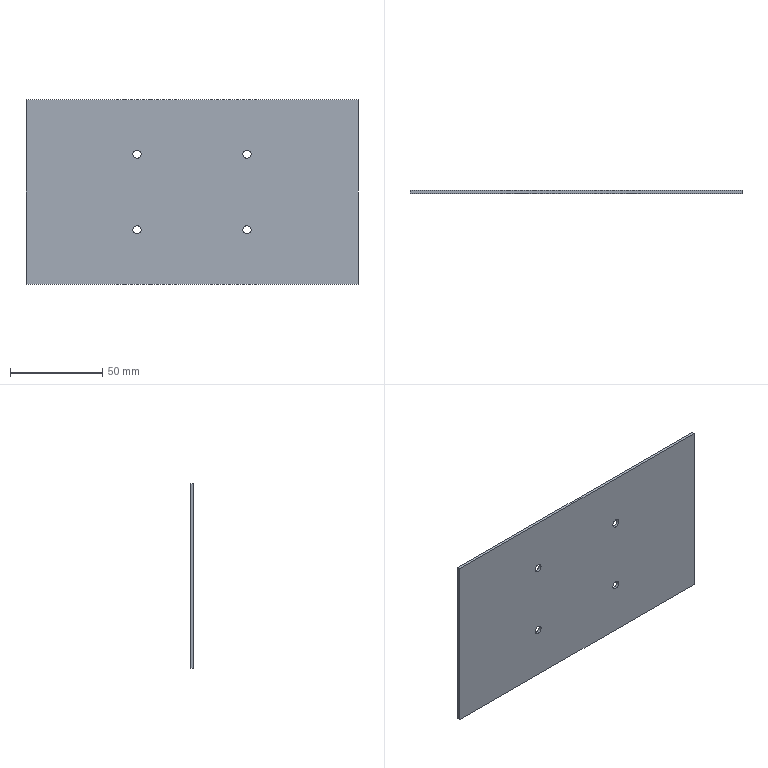Component | SolidWorks | CopperGasket-1 | 1 solid | 14 faces | box 180 x 1.5 x 100.27 mm | volume 26975 mm3 | cylinder 8 | plane 6 | commonest cylinder face diameters 4.542 x8
build123d program:
from build123d import *

# Parameters (mm, degrees)
SKETCH1_W               = 100.269
SKETCH1_H               = 180
BOSS_EXTRUDE1_DEPTH     = 1.5
SKETCH3_W               = 55.775
SKETCH3_H               = 106
BOSS_EXTRUDE2_DEPTH     = 1.5
CUT_EXTRUDE1_DEPTH      = 158.947
CUT_EXTRUDE1_DEPTH_BACK = 158.947
SKETCH2_R               = 2.271


with BuildPart() as part:
    # Sketch1 → Boss-Extrude1 (new body)
    with BuildSketch(Plane.XY):
        with Locations((0, -59.772)):
            Rectangle(SKETCH1_W, SKETCH1_H)
    extrude(amount=BOSS_EXTRUDE1_DEPTH)


with BuildPart() as body_2:
    # Sketch3 → Boss-Extrude2 (new body)
    with BuildSketch(Plane.XY.offset(1.5)):
        with Locations((0, -53)):
            Rectangle(SKETCH3_W, SKETCH3_H)
    extrude(amount=-BOSS_EXTRUDE2_DEPTH)


with BuildPart() as cut_extrude1_tool:
    # Sketch2 → Cut-Extrude1 (new, two sides: drawn at the far end of the back side and taken through both)
    with BuildSketch(Plane.XY.offset(1.5).offset(-CUT_EXTRUDE1_DEPTH_BACK)):
        with Locations((20.473, -29.973)):
            Circle(SKETCH2_R)
        with Locations((20.473, -89.571)):
            Circle(SKETCH2_R)
        with Locations((-20.473, -29.973)):
            Circle(SKETCH2_R)
        with Locations((-20.473, -89.571)):
            Circle(SKETCH2_R)
    extrude(amount=CUT_EXTRUDE1_DEPTH + CUT_EXTRUDE1_DEPTH_BACK)


with BuildPart() as part_1:
    add(part.part)

    # Cut-Extrude1: cut by cut_extrude1_tool
    add(cut_extrude1_tool.part, mode=Mode.SUBTRACT)


with BuildPart() as body_2_1:
    add(body_2.part)

    # Cut-Extrude1: cut by cut_extrude1_tool
    add(cut_extrude1_tool.part, mode=Mode.SUBTRACT)


with BuildPart() as part_2:
    add(part_1.part)

    # Combine2: union body 2
    add(body_2_1.part)


solid = part_2.part

# Placed as in the assembly
solid = solid.moved(Location((-3, 96.74, 0), (90, 0, 90)))
STEP:
#1=CARTESIAN_POINT('',(1.062,3.75,-0.7166));
#2=VERTEX_POINT('',#1);
#3=CARTESIAN_POINT('',(1.062,3.75,-0.8954));
#4=VERTEX_POINT('',#3);
#5=CARTESIAN_POINT('',(1.062,3.75,-0.806));
#6=DIRECTION('',(0.,1.,0.));
#7=DIRECTION('',(0.,0.,-1.));
#8=AXIS2_PLACEMENT_3D('',#5,#6,#7);
#9=CIRCLE('',#8,0.08941);
#10=EDGE_CURVE('',#2,#4,#9,.T.);
#11=ORIENTED_EDGE('',*,*,#10,.F.);
#12=CARTESIAN_POINT('',(1.062,3.809,-0.7166));
#13=VERTEX_POINT('',#12);
#14=CARTESIAN_POINT('',(1.062,3.75,-0.7166));
#15=DIRECTION('',(0.,1.,0.));
#16=VECTOR('',#15,39.37);
#17=LINE('',#14,#16);
#18=EDGE_CURVE('',#2,#13,#17,.T.);
#19=ORIENTED_EDGE('',*,*,#18,.T.);
#20=CARTESIAN_POINT('',(1.062,3.809,-0.8954));
#21=VERTEX_POINT('',#20);
#22=CARTESIAN_POINT('',(1.062,3.809,-0.7166));
#23=CARTESIAN_POINT('',(1.074,3.809,-0.7166));
#24=CARTESIAN_POINT('',(1.085,3.809,-0.7189));
#25=CARTESIAN_POINT('',(1.107,3.809,-0.7279));
#26=CARTESIAN_POINT('',(1.117,3.809,-0.7345));
#27=CARTESIAN_POINT('',(1.133,3.809,-0.7511));
#28=CARTESIAN_POINT('',(1.14,3.809,-0.761));
#29=CARTESIAN_POINT('',(1.149,3.809,-0.7826));
#30=CARTESIAN_POINT('',(1.151,3.809,-0.7943));
#31=CARTESIAN_POINT('',(1.151,3.809,-0.8177));
#32=CARTESIAN_POINT('',(1.149,3.809,-0.8294));
#33=CARTESIAN_POINT('',(1.14,3.809,-0.8511));
#34=CARTESIAN_POINT('',(1.133,3.809,-0.861));
#35=CARTESIAN_POINT('',(1.117,3.809,-0.8775));
#36=CARTESIAN_POINT('',(1.107,3.809,-0.8842));
#37=CARTESIAN_POINT('',(1.085,3.809,-0.8931));
#38=CARTESIAN_POINT('',(1.074,3.809,-0.8954));
#39=CARTESIAN_POINT('',(1.062,3.809,-0.8954));
#40=B_SPLINE_CURVE_WITH_KNOTS('',3,(#22,#23,#24,#25,#26,#27,#28,#29,#30,#31,#32,#33,#34,#35,#36,#37,#38,#39),.UNSPECIFIED.,.F.,.F.,(4,2,2,2,2,2,2,2,4),(0.5,0.5625,0.625,0.6875,0.75,0.8125,0.875,0.9375,1.),.UNSPECIFIED.);
#41=EDGE_CURVE('',#13,#21,#40,.T.);
#42=ORIENTED_EDGE('',*,*,#41,.T.);
#43=CARTESIAN_POINT('',(1.062,3.75,-0.8954));
#44=DIRECTION('',(0.,1.,0.));
#45=VECTOR('',#44,39.37);
#46=LINE('',#43,#45);
#47=EDGE_CURVE('',#4,#21,#46,.T.);
#48=ORIENTED_EDGE('',*,*,#47,.F.);
#49=EDGE_LOOP('',(#11,#19,#42,#48));
#50=FACE_OUTER_BOUND('',#49,.T.);
#51=CARTESIAN_POINT('',(1.062,3.75,-0.806));
#52=DIRECTION('',(0.,1.,0.));
#53=DIRECTION('',(0.,0.,-1.));
#54=AXIS2_PLACEMENT_3D('',#51,#52,#53);
#55=CYLINDRICAL_SURFACE('',#54,0.08941);
#56=ADVANCED_FACE('',(#50),#55,.F.);
#57=CARTESIAN_POINT('',(3.408,3.75,-0.7166));
#58=VERTEX_POINT('',#57);
#59=CARTESIAN_POINT('',(3.408,3.75,-0.8954));
#60=VERTEX_POINT('',#59);
#61=CARTESIAN_POINT('',(3.408,3.75,-0.806));
#62=DIRECTION('',(0.,1.,0.));
#63=DIRECTION('',(0.,0.,-1.));
#64=AXIS2_PLACEMENT_3D('',#61,#62,#63);
#65=CIRCLE('',#64,0.08941);
#66=EDGE_CURVE('',#58,#60,#65,.T.);
#67=ORIENTED_EDGE('',*,*,#66,.F.);
#68=CARTESIAN_POINT('',(3.408,3.809,-0.7166));
#69=VERTEX_POINT('',#68);
#70=CARTESIAN_POINT('',(3.408,3.75,-0.7166));
#71=DIRECTION('',(0.,1.,0.));
#72=VECTOR('',#71,39.37);
#73=LINE('',#70,#72);
#74=EDGE_CURVE('',#58,#69,#73,.T.);
#75=ORIENTED_EDGE('',*,*,#74,.T.);
#76=CARTESIAN_POINT('',(3.408,3.809,-0.8954));
#77=VERTEX_POINT('',#76);
#78=CARTESIAN_POINT('',(3.408,3.809,-0.7166));
#79=CARTESIAN_POINT('',(3.42,3.809,-0.7166));
#80=CARTESIAN_POINT('',(3.432,3.809,-0.7189));
#81=CARTESIAN_POINT('',(3.453,3.809,-0.7279));
#82=CARTESIAN_POINT('',(3.463,3.809,-0.7345));
#83=CARTESIAN_POINT('',(3.48,3.809,-0.7511));
#84=CARTESIAN_POINT('',(3.486,3.809,-0.761));
#85=CARTESIAN_POINT('',(3.495,3.809,-0.7826));
#86=CARTESIAN_POINT('',(3.498,3.809,-0.7943));
#87=CARTESIAN_POINT('',(3.498,3.809,-0.8177));
#88=CARTESIAN_POINT('',(3.495,3.809,-0.8294));
#89=CARTESIAN_POINT('',(3.486,3.809,-0.8511));
#90=CARTESIAN_POINT('',(3.48,3.809,-0.861));
#91=CARTESIAN_POINT('',(3.463,3.809,-0.8775));
#92=CARTESIAN_POINT('',(3.453,3.809,-0.8842));
#93=CARTESIAN_POINT('',(3.432,3.809,-0.8931));
#94=CARTESIAN_POINT('',(3.42,3.809,-0.8954));
#95=CARTESIAN_POINT('',(3.408,3.809,-0.8954));
#96=B_SPLINE_CURVE_WITH_KNOTS('',3,(#78,#79,#80,#81,#82,#83,#84,#85,#86,#87,#88,#89,#90,#91,#92,#93,#94,#95),.UNSPECIFIED.,.F.,.F.,(4,2,2,2,2,2,2,2,4),(0.5,0.5625,0.625,0.6875,0.75,0.8125,0.875,0.9375,1.),.UNSPECIFIED.);
#97=EDGE_CURVE('',#69,#77,#96,.T.);
#98=ORIENTED_EDGE('',*,*,#97,.T.);
#99=CARTESIAN_POINT('',(3.408,3.75,-0.8954));
#100=DIRECTION('',(0.,1.,0.));
#101=VECTOR('',#100,39.37);
#102=LINE('',#99,#101);
#103=EDGE_CURVE('',#60,#77,#102,.T.);
#104=ORIENTED_EDGE('',*,*,#103,.F.);
#105=EDGE_LOOP('',(#67,#75,#98,#104));
#106=FACE_OUTER_BOUND('',#105,.T.);
#107=CARTESIAN_POINT('',(3.408,3.75,-0.806));
#108=DIRECTION('',(0.,1.,0.));
#109=DIRECTION('',(0.,0.,-1.));
#110=AXIS2_PLACEMENT_3D('',#107,#108,#109);
#111=CYLINDRICAL_SURFACE('',#110,0.08941);
#112=ADVANCED_FACE('',(#106),#111,.F.);
#113=CARTESIAN_POINT('',(1.062,3.75,0.8954));
#114=VERTEX_POINT('',#113);
#115=CARTESIAN_POINT('',(1.062,3.75,0.7166));
#116=VERTEX_POINT('',#115);
#117=CARTESIAN_POINT('',(1.062,3.75,0.806));
#118=DIRECTION('',(0.,1.,0.));
#119=DIRECTION('',(0.,0.,-1.));
#120=AXIS2_PLACEMENT_3D('',#117,#118,#119);
#121=CIRCLE('',#120,0.08941);
#122=EDGE_CURVE('',#114,#116,#121,.T.);
#123=ORIENTED_EDGE('',*,*,#122,.F.);
#124=CARTESIAN_POINT('',(1.062,3.809,0.8954));
#125=VERTEX_POINT('',#124);
#126=CARTESIAN_POINT('',(1.062,3.75,0.8954));
#127=DIRECTION('',(0.,1.,0.));
#128=VECTOR('',#127,39.37);
#129=LINE('',#126,#128);
#130=EDGE_CURVE('',#114,#125,#129,.T.);
#131=ORIENTED_EDGE('',*,*,#130,.T.);
#132=CARTESIAN_POINT('',(1.062,3.809,0.7166));
#133=VERTEX_POINT('',#132);
#134=CARTESIAN_POINT('',(1.062,3.809,0.8954));
#135=CARTESIAN_POINT('',(1.074,3.809,0.8954));
#136=CARTESIAN_POINT('',(1.085,3.809,0.8931));
#137=CARTESIAN_POINT('',(1.107,3.809,0.8842));
#138=CARTESIAN_POINT('',(1.117,3.809,0.8775));
#139=CARTESIAN_POINT('',(1.133,3.809,0.861));
#140=CARTESIAN_POINT('',(1.14,3.809,0.8511));
#141=CARTESIAN_POINT('',(1.149,3.809,0.8294));
#142=CARTESIAN_POINT('',(1.151,3.809,0.8177));
#143=CARTESIAN_POINT('',(1.151,3.809,0.7943));
#144=CARTESIAN_POINT('',(1.149,3.809,0.7826));
#145=CARTESIAN_POINT('',(1.14,3.809,0.761));
#146=CARTESIAN_POINT('',(1.133,3.809,0.7511));
#147=CARTESIAN_POINT('',(1.117,3.809,0.7345));
#148=CARTESIAN_POINT('',(1.107,3.809,0.7279));
#149=CARTESIAN_POINT('',(1.085,3.809,0.7189));
#150=CARTESIAN_POINT('',(1.074,3.809,0.7166));
#151=CARTESIAN_POINT('',(1.062,3.809,0.7166));
#152=B_SPLINE_CURVE_WITH_KNOTS('',3,(#134,#135,#136,#137,#138,#139,#140,#141,#142,#143,#144,#145,#146,#147,#148,#149,#150,#151),.UNSPECIFIED.,.F.,.F.,(4,2,2,2,2,2,2,2,4),(0.5,0.5625,0.625,0.6875,0.75,0.8125,0.875,0.9375,1.),.UNSPECIFIED.);
#153=EDGE_CURVE('',#125,#133,#152,.T.);
#154=ORIENTED_EDGE('',*,*,#153,.T.);
#155=CARTESIAN_POINT('',(1.062,3.75,0.7166));
#156=DIRECTION('',(0.,1.,0.));
#157=VECTOR('',#156,39.37);
#158=LINE('',#155,#157);
#159=EDGE_CURVE('',#116,#133,#158,.T.);
#160=ORIENTED_EDGE('',*,*,#159,.F.);
#161=EDGE_LOOP('',(#123,#131,#154,#160));
#162=FACE_OUTER_BOUND('',#161,.T.);
#163=CARTESIAN_POINT('',(1.062,3.75,0.806));
#164=DIRECTION('',(0.,1.,0.));
#165=DIRECTION('',(0.,0.,-1.));
#166=AXIS2_PLACEMENT_3D('',#163,#164,#165);
#167=CYLINDRICAL_SURFACE('',#166,0.08941);
#168=ADVANCED_FACE('',(#162),#167,.F.);
#169=CARTESIAN_POINT('',(3.408,3.75,0.8954));
#170=VERTEX_POINT('',#169);
#171=CARTESIAN_POINT('',(3.408,3.75,0.7166));
#172=VERTEX_POINT('',#171);
#173=CARTESIAN_POINT('',(3.408,3.75,0.806));
#174=DIRECTION('',(0.,1.,0.));
#175=DIRECTION('',(0.,0.,-1.));
#176=AXIS2_PLACEMENT_3D('',#173,#174,#175);
#177=CIRCLE('',#176,0.08941);
#178=EDGE_CURVE('',#170,#172,#177,.T.);
#179=ORIENTED_EDGE('',*,*,#178,.F.);
#180=CARTESIAN_POINT('',(3.408,3.809,0.8954));
#181=VERTEX_POINT('',#180);
#182=CARTESIAN_POINT('',(3.408,3.75,0.8954));
#183=DIRECTION('',(0.,1.,0.));
#184=VECTOR('',#183,39.37);
#185=LINE('',#182,#184);
#186=EDGE_CURVE('',#170,#181,#185,.T.);
#187=ORIENTED_EDGE('',*,*,#186,.T.);
#188=CARTESIAN_POINT('',(3.408,3.809,0.7166));
#189=VERTEX_POINT('',#188);
#190=CARTESIAN_POINT('',(3.408,3.809,0.8954));
#191=CARTESIAN_POINT('',(3.42,3.809,0.8954));
#192=CARTESIAN_POINT('',(3.432,3.809,0.8931));
#193=CARTESIAN_POINT('',(3.453,3.809,0.8842));
#194=CARTESIAN_POINT('',(3.463,3.809,0.8775));
#195=CARTESIAN_POINT('',(3.48,3.809,0.861));
#196=CARTESIAN_POINT('',(3.486,3.809,0.8511));
#197=CARTESIAN_POINT('',(3.495,3.809,0.8294));
#198=CARTESIAN_POINT('',(3.498,3.809,0.8177));
#199=CARTESIAN_POINT('',(3.498,3.809,0.7943));
#200=CARTESIAN_POINT('',(3.495,3.809,0.7826));
#201=CARTESIAN_POINT('',(3.486,3.809,0.761));
#202=CARTESIAN_POINT('',(3.48,3.809,0.7511));
#203=CARTESIAN_POINT('',(3.463,3.809,0.7345));
#204=CARTESIAN_POINT('',(3.453,3.809,0.7279));
#205=CARTESIAN_POINT('',(3.432,3.809,0.7189));
#206=CARTESIAN_POINT('',(3.42,3.809,0.7166));
#207=CARTESIAN_POINT('',(3.408,3.809,0.7166));
#208=B_SPLINE_CURVE_WITH_KNOTS('',3,(#190,#191,#192,#193,#194,#195,#196,#197,#198,#199,#200,#201,#202,#203,#204,#205,#206,#207),.UNSPECIFIED.,.F.,.F.,(4,2,2,2,2,2,2,2,4),(0.5,0.5625,0.625,0.6875,0.75,0.8125,0.875,0.9375,1.),.UNSPECIFIED.);
#209=EDGE_CURVE('',#181,#189,#208,.T.);
#210=ORIENTED_EDGE('',*,*,#209,.T.);
#211=CARTESIAN_POINT('',(3.408,3.75,0.7166));
#212=DIRECTION('',(0.,1.,0.));
#213=VECTOR('',#212,39.37);
#214=LINE('',#211,#213);
#215=EDGE_CURVE('',#172,#189,#214,.T.);
#216=ORIENTED_EDGE('',*,*,#215,.F.);
#217=EDGE_LOOP('',(#179,#187,#210,#216));
#218=FACE_OUTER_BOUND('',#217,.T.);
#219=CARTESIAN_POINT('',(3.408,3.75,0.806));
#220=DIRECTION('',(0.,1.,0.));
#221=DIRECTION('',(0.,0.,-1.));
#222=AXIS2_PLACEMENT_3D('',#219,#220,#221);
#223=CYLINDRICAL_SURFACE('',#222,0.08941);
#224=ADVANCED_FACE('',(#218),#223,.F.);
#225=CARTESIAN_POINT('',(5.778,3.75,-1.974));
#226=VERTEX_POINT('',#225);
#227=CARTESIAN_POINT('',(-1.308,3.75,-1.974));
#228=VERTEX_POINT('',#227);
#229=CARTESIAN_POINT('',(5.778,3.75,-1.974));
#230=DIRECTION('',(-1.,-0.,0.));
#231=VECTOR('',#230,39.37);
#232=LINE('',#229,#231);
#233=EDGE_CURVE('',#226,#228,#232,.T.);
#234=ORIENTED_EDGE('',*,*,#233,.T.);
#235=CARTESIAN_POINT('',(-1.308,3.809,-1.974));
#236=VERTEX_POINT('',#235);
#237=CARTESIAN_POINT('',(-1.308,3.809,-1.974));
#238=DIRECTION('',(0.,-1.,-0.));
#239=VECTOR('',#238,39.37);
#240=LINE('',#237,#239);
#241=EDGE_CURVE('',#236,#228,#240,.T.);
#242=ORIENTED_EDGE('',*,*,#241,.F.);
#243=CARTESIAN_POINT('',(5.778,3.809,-1.974));
#244=VERTEX_POINT('',#243);
#245=CARTESIAN_POINT('',(5.778,3.809,-1.974));
#246=DIRECTION('',(-1.,-0.,0.));
#247=VECTOR('',#246,39.37);
#248=LINE('',#245,#247);
#249=EDGE_CURVE('',#244,#236,#248,.T.);
#250=ORIENTED_EDGE('',*,*,#249,.F.);
#251=CARTESIAN_POINT('',(5.778,3.809,-1.974));
#252=DIRECTION('',(0.,-1.,-0.));
#253=VECTOR('',#252,39.37);
#254=LINE('',#251,#253);
#255=EDGE_CURVE('',#244,#226,#254,.T.);
#256=ORIENTED_EDGE('',*,*,#255,.T.);
#257=EDGE_LOOP('',(#234,#242,#250,#256));
#258=FACE_OUTER_BOUND('',#257,.T.);
#259=CARTESIAN_POINT('',(5.778,3.809,-1.974));
#260=DIRECTION('',(0.,-0.,1.));
#261=DIRECTION('',(1.,0.,-0.));
#262=AXIS2_PLACEMENT_3D('',#259,#260,#261);
#263=PLANE('',#262);
#264=ADVANCED_FACE('',(#258),#263,.F.);
#265=CARTESIAN_POINT('',(-1.308,3.75,1.974));
#266=VERTEX_POINT('',#265);
#267=CARTESIAN_POINT('',(-1.308,3.75,-1.974));
#268=DIRECTION('',(0.,-0.,1.));
#269=VECTOR('',#268,39.37);
#270=LINE('',#267,#269);
#271=EDGE_CURVE('',#228,#266,#270,.T.);
#272=ORIENTED_EDGE('',*,*,#271,.T.);
#273=CARTESIAN_POINT('',(-1.308,3.809,1.974));
#274=VERTEX_POINT('',#273);
#275=CARTESIAN_POINT('',(-1.308,3.809,1.974));
#276=DIRECTION('',(0.,-1.,-0.));
#277=VECTOR('',#276,39.37);
#278=LINE('',#275,#277);
#279=EDGE_CURVE('',#274,#266,#278,.T.);
#280=ORIENTED_EDGE('',*,*,#279,.F.);
#281=CARTESIAN_POINT('',(-1.308,3.809,-1.974));
#282=DIRECTION('',(0.,-0.,1.));
#283=VECTOR('',#282,39.37);
#284=LINE('',#281,#283);
#285=EDGE_CURVE('',#236,#274,#284,.T.);
#286=ORIENTED_EDGE('',*,*,#285,.F.);
#287=ORIENTED_EDGE('',*,*,#241,.T.);
#288=EDGE_LOOP('',(#272,#280,#286,#287));
#289=FACE_OUTER_BOUND('',#288,.T.);
#290=CARTESIAN_POINT('',(-1.308,3.809,-1.974));
#291=DIRECTION('',(1.,0.,-0.));
#292=DIRECTION('',(0.,-1.,-0.));
#293=AXIS2_PLACEMENT_3D('',#290,#291,#292);
#294=PLANE('',#293);
#295=ADVANCED_FACE('',(#289),#294,.F.);
#296=CARTESIAN_POINT('',(5.778,3.75,1.974));
#297=VERTEX_POINT('',#296);
#298=CARTESIAN_POINT('',(-1.308,3.75,1.974));
#299=DIRECTION('',(1.,0.,-0.));
#300=VECTOR('',#299,39.37);
#301=LINE('',#298,#300);
#302=EDGE_CURVE('',#266,#297,#301,.T.);
#303=ORIENTED_EDGE('',*,*,#302,.T.);
#304=CARTESIAN_POINT('',(5.778,3.809,1.974));
#305=VERTEX_POINT('',#304);
#306=CARTESIAN_POINT('',(5.778,3.809,1.974));
#307=DIRECTION('',(0.,-1.,-0.));
#308=VECTOR('',#307,39.37);
#309=LINE('',#306,#308);
#310=EDGE_CURVE('',#305,#297,#309,.T.);
#311=ORIENTED_EDGE('',*,*,#310,.F.);
#312=CARTESIAN_POINT('',(-1.308,3.809,1.974));
#313=DIRECTION('',(1.,0.,-0.));
#314=VECTOR('',#313,39.37);
#315=LINE('',#312,#314);
#316=EDGE_CURVE('',#274,#305,#315,.T.);
#317=ORIENTED_EDGE('',*,*,#316,.F.);
#318=ORIENTED_EDGE('',*,*,#279,.T.);
#319=EDGE_LOOP('',(#303,#311,#317,#318));
#320=FACE_OUTER_BOUND('',#319,.T.);
#321=CARTESIAN_POINT('',(-1.308,3.809,1.974));
#322=DIRECTION('',(-0.,0.,-1.));
#323=DIRECTION('',(-1.,-0.,0.));
#324=AXIS2_PLACEMENT_3D('',#321,#322,#323);
#325=PLANE('',#324);
#326=ADVANCED_FACE('',(#320),#325,.F.);
#327=CARTESIAN_POINT('',(5.778,3.75,1.974));
#328=DIRECTION('',(0.,0.,-1.));
#329=VECTOR('',#328,39.37);
#330=LINE('',#327,#329);
#331=EDGE_CURVE('',#297,#226,#330,.T.);
#332=ORIENTED_EDGE('',*,*,#331,.T.);
#333=ORIENTED_EDGE('',*,*,#255,.F.);
#334=CARTESIAN_POINT('',(5.778,3.809,1.974));
#335=DIRECTION('',(0.,0.,-1.));
#336=VECTOR('',#335,39.37);
#337=LINE('',#334,#336);
#338=EDGE_CURVE('',#305,#244,#337,.T.);
#339=ORIENTED_EDGE('',*,*,#338,.F.);
#340=ORIENTED_EDGE('',*,*,#310,.T.);
#341=EDGE_LOOP('',(#332,#333,#339,#340));
#342=FACE_OUTER_BOUND('',#341,.T.);
#343=CARTESIAN_POINT('',(5.778,3.809,1.974));
#344=DIRECTION('',(-1.,-0.,0.));
#345=DIRECTION('',(0.,1.,0.));
#346=AXIS2_PLACEMENT_3D('',#343,#344,#345);
#347=PLANE('',#346);
#348=ADVANCED_FACE('',(#342),#347,.F.);
#349=CARTESIAN_POINT('',(1.062,3.809,-0.8954));
#350=CARTESIAN_POINT('',(1.05,3.809,-0.8954));
#351=CARTESIAN_POINT('',(1.039,3.809,-0.8931));
#352=CARTESIAN_POINT('',(1.017,3.809,-0.8842));
#353=CARTESIAN_POINT('',(1.007,3.809,-0.8775));
#354=CARTESIAN_POINT('',(0.9904,3.809,-0.861));
#355=CARTESIAN_POINT('',(0.9838,3.809,-0.8511));
#356=CARTESIAN_POINT('',(0.9748,3.809,-0.8294));
#357=CARTESIAN_POINT('',(0.9725,3.809,-0.8177));
#358=CARTESIAN_POINT('',(0.9725,3.809,-0.7943));
#359=CARTESIAN_POINT('',(0.9748,3.809,-0.7826));
#360=CARTESIAN_POINT('',(0.9838,3.809,-0.761));
#361=CARTESIAN_POINT('',(0.9904,3.809,-0.7511));
#362=CARTESIAN_POINT('',(1.007,3.809,-0.7345));
#363=CARTESIAN_POINT('',(1.017,3.809,-0.7279));
#364=CARTESIAN_POINT('',(1.039,3.809,-0.7189));
#365=CARTESIAN_POINT('',(1.05,3.809,-0.7166));
#366=CARTESIAN_POINT('',(1.062,3.809,-0.7166));
#367=B_SPLINE_CURVE_WITH_KNOTS('',3,(#349,#350,#351,#352,#353,#354,#355,#356,#357,#358,#359,#360,#361,#362,#363,#364,#365,#366),.UNSPECIFIED.,.F.,.F.,(4,2,2,2,2,2,2,2,4),(0.,0.0625,0.125,0.1875,0.25,0.3125,0.375,0.4375,0.5),.UNSPECIFIED.);
#368=EDGE_CURVE('',#21,#13,#367,.T.);
#369=ORIENTED_EDGE('',*,*,#368,.F.);
#370=ORIENTED_EDGE('',*,*,#41,.F.);
#371=EDGE_LOOP('',(#369,#370));
#372=FACE_BOUND('',#371,.T.);
#373=CARTESIAN_POINT('',(3.408,3.809,-0.8954));
#374=CARTESIAN_POINT('',(3.397,3.809,-0.8954));
#375=CARTESIAN_POINT('',(3.385,3.809,-0.8931));
#376=CARTESIAN_POINT('',(3.363,3.809,-0.8842));
#377=CARTESIAN_POINT('',(3.353,3.809,-0.8775));
#378=CARTESIAN_POINT('',(3.337,3.809,-0.861));
#379=CARTESIAN_POINT('',(3.33,3.809,-0.8511));
#380=CARTESIAN_POINT('',(3.321,3.809,-0.8294));
#381=CARTESIAN_POINT('',(3.319,3.809,-0.8177));
#382=CARTESIAN_POINT('',(3.319,3.809,-0.7943));
#383=CARTESIAN_POINT('',(3.321,3.809,-0.7826));
#384=CARTESIAN_POINT('',(3.33,3.809,-0.761));
#385=CARTESIAN_POINT('',(3.337,3.809,-0.7511));
#386=CARTESIAN_POINT('',(3.353,3.809,-0.7345));
#387=CARTESIAN_POINT('',(3.363,3.809,-0.7279));
#388=CARTESIAN_POINT('',(3.385,3.809,-0.7189));
#389=CARTESIAN_POINT('',(3.397,3.809,-0.7166));
#390=CARTESIAN_POINT('',(3.408,3.809,-0.7166));
#391=B_SPLINE_CURVE_WITH_KNOTS('',3,(#373,#374,#375,#376,#377,#378,#379,#380,#381,#382,#383,#384,#385,#386,#387,#388,#389,#390),.UNSPECIFIED.,.F.,.F.,(4,2,2,2,2,2,2,2,4),(0.,0.0625,0.125,0.1875,0.25,0.3125,0.375,0.4375,0.5),.UNSPECIFIED.);
#392=EDGE_CURVE('',#77,#69,#391,.T.);
#393=ORIENTED_EDGE('',*,*,#392,.F.);
#394=ORIENTED_EDGE('',*,*,#97,.F.);
#395=EDGE_LOOP('',(#393,#394));
#396=FACE_BOUND('',#395,.T.);
#397=CARTESIAN_POINT('',(1.062,3.809,0.7166));
#398=CARTESIAN_POINT('',(1.05,3.809,0.7166));
#399=CARTESIAN_POINT('',(1.039,3.809,0.7189));
#400=CARTESIAN_POINT('',(1.017,3.809,0.7279));
#401=CARTESIAN_POINT('',(1.007,3.809,0.7345));
#402=CARTESIAN_POINT('',(0.9904,3.809,0.7511));
#403=CARTESIAN_POINT('',(0.9838,3.809,0.761));
#404=CARTESIAN_POINT('',(0.9748,3.809,0.7826));
#405=CARTESIAN_POINT('',(0.9725,3.809,0.7943));
#406=CARTESIAN_POINT('',(0.9725,3.809,0.8177));
#407=CARTESIAN_POINT('',(0.9748,3.809,0.8294));
#408=CARTESIAN_POINT('',(0.9838,3.809,0.8511));
#409=CARTESIAN_POINT('',(0.9904,3.809,0.861));
#410=CARTESIAN_POINT('',(1.007,3.809,0.8775));
#411=CARTESIAN_POINT('',(1.017,3.809,0.8842));
#412=CARTESIAN_POINT('',(1.039,3.809,0.8931));
#413=CARTESIAN_POINT('',(1.05,3.809,0.8954));
#414=CARTESIAN_POINT('',(1.062,3.809,0.8954));
#415=B_SPLINE_CURVE_WITH_KNOTS('',3,(#397,#398,#399,#400,#401,#402,#403,#404,#405,#406,#407,#408,#409,#410,#411,#412,#413,#414),.UNSPECIFIED.,.F.,.F.,(4,2,2,2,2,2,2,2,4),(0.,0.0625,0.125,0.1875,0.25,0.3125,0.375,0.4375,0.5),.UNSPECIFIED.);
#416=EDGE_CURVE('',#133,#125,#415,.T.);
#417=ORIENTED_EDGE('',*,*,#416,.F.);
#418=ORIENTED_EDGE('',*,*,#153,.F.);
#419=EDGE_LOOP('',(#417,#418));
#420=FACE_BOUND('',#419,.T.);
#421=CARTESIAN_POINT('',(3.408,3.809,0.7166));
#422=CARTESIAN_POINT('',(3.397,3.809,0.7166));
#423=CARTESIAN_POINT('',(3.385,3.809,0.7189));
#424=CARTESIAN_POINT('',(3.363,3.809,0.7279));
#425=CARTESIAN_POINT('',(3.353,3.809,0.7345));
#426=CARTESIAN_POINT('',(3.337,3.809,0.7511));
#427=CARTESIAN_POINT('',(3.33,3.809,0.761));
#428=CARTESIAN_POINT('',(3.321,3.809,0.7826));
#429=CARTESIAN_POINT('',(3.319,3.809,0.7943));
#430=CARTESIAN_POINT('',(3.319,3.809,0.8177));
#431=CARTESIAN_POINT('',(3.321,3.809,0.8294));
#432=CARTESIAN_POINT('',(3.33,3.809,0.8511));
#433=CARTESIAN_POINT('',(3.337,3.809,0.861));
#434=CARTESIAN_POINT('',(3.353,3.809,0.8775));
#435=CARTESIAN_POINT('',(3.363,3.809,0.8842));
#436=CARTESIAN_POINT('',(3.385,3.809,0.8931));
#437=CARTESIAN_POINT('',(3.397,3.809,0.8954));
#438=CARTESIAN_POINT('',(3.408,3.809,0.8954));
#439=B_SPLINE_CURVE_WITH_KNOTS('',3,(#421,#422,#423,#424,#425,#426,#427,#428,#429,#430,#431,#432,#433,#434,#435,#436,#437,#438),.UNSPECIFIED.,.F.,.F.,(4,2,2,2,2,2,2,2,4),(0.,0.0625,0.125,0.1875,0.25,0.3125,0.375,0.4375,0.5),.UNSPECIFIED.);
#440=EDGE_CURVE('',#189,#181,#439,.T.);
#441=ORIENTED_EDGE('',*,*,#440,.F.);
#442=ORIENTED_EDGE('',*,*,#209,.F.);
#443=EDGE_LOOP('',(#441,#442));
#444=FACE_BOUND('',#443,.T.);
#445=ORIENTED_EDGE('',*,*,#249,.T.);
#446=ORIENTED_EDGE('',*,*,#285,.T.);
#447=ORIENTED_EDGE('',*,*,#316,.T.);
#448=ORIENTED_EDGE('',*,*,#338,.T.);
#449=EDGE_LOOP('',(#445,#446,#447,#448));
#450=FACE_OUTER_BOUND('',#449,.T.);
#451=CARTESIAN_POINT('',(-0.1181,3.809,-0.));
#452=DIRECTION('',(0.,1.,0.));
#453=DIRECTION('',(0.,0.,-1.));
#454=AXIS2_PLACEMENT_3D('',#451,#452,#453);
#455=PLANE('',#454);
#456=ADVANCED_FACE('',(#372,#396,#420,#444,#450),#455,.T.);
#457=CARTESIAN_POINT('',(1.062,3.75,-0.806));
#458=DIRECTION('',(0.,1.,0.));
#459=DIRECTION('',(0.,0.,-1.));
#460=AXIS2_PLACEMENT_3D('',#457,#458,#459);
#461=CIRCLE('',#460,0.08941);
#462=EDGE_CURVE('',#4,#2,#461,.T.);
#463=ORIENTED_EDGE('',*,*,#462,.T.);
#464=ORIENTED_EDGE('',*,*,#10,.T.);
#465=EDGE_LOOP('',(#463,#464));
#466=FACE_BOUND('',#465,.T.);
#467=CARTESIAN_POINT('',(3.408,3.75,-0.806));
#468=DIRECTION('',(0.,1.,0.));
#469=DIRECTION('',(0.,0.,-1.));
#470=AXIS2_PLACEMENT_3D('',#467,#468,#469);
#471=CIRCLE('',#470,0.08941);
#472=EDGE_CURVE('',#60,#58,#471,.T.);
#473=ORIENTED_EDGE('',*,*,#472,.T.);
#474=ORIENTED_EDGE('',*,*,#66,.T.);
#475=EDGE_LOOP('',(#473,#474));
#476=FACE_BOUND('',#475,.T.);
#477=CARTESIAN_POINT('',(1.062,3.75,0.806));
#478=DIRECTION('',(0.,1.,0.));
#479=DIRECTION('',(0.,0.,-1.));
#480=AXIS2_PLACEMENT_3D('',#477,#478,#479);
#481=CIRCLE('',#480,0.08941);
#482=EDGE_CURVE('',#116,#114,#481,.T.);
#483=ORIENTED_EDGE('',*,*,#482,.T.);
#484=ORIENTED_EDGE('',*,*,#122,.T.);
#485=EDGE_LOOP('',(#483,#484));
#486=FACE_BOUND('',#485,.T.);
#487=CARTESIAN_POINT('',(3.408,3.75,0.806));
#488=DIRECTION('',(0.,1.,0.));
#489=DIRECTION('',(0.,0.,-1.));
#490=AXIS2_PLACEMENT_3D('',#487,#488,#489);
#491=CIRCLE('',#490,0.08941);
#492=EDGE_CURVE('',#172,#170,#491,.T.);
#493=ORIENTED_EDGE('',*,*,#492,.T.);
#494=ORIENTED_EDGE('',*,*,#178,.T.);
#495=EDGE_LOOP('',(#493,#494));
#496=FACE_BOUND('',#495,.T.);
#497=ORIENTED_EDGE('',*,*,#233,.F.);
#498=ORIENTED_EDGE('',*,*,#331,.F.);
#499=ORIENTED_EDGE('',*,*,#302,.F.);
#500=ORIENTED_EDGE('',*,*,#271,.F.);
#501=EDGE_LOOP('',(#497,#498,#499,#500));
#502=FACE_OUTER_BOUND('',#501,.T.);
#503=CARTESIAN_POINT('',(-0.1181,3.75,-0.));
#504=DIRECTION('',(0.,1.,0.));
#505=DIRECTION('',(0.,0.,-1.));
#506=AXIS2_PLACEMENT_3D('',#503,#504,#505);
#507=PLANE('',#506);
#508=ADVANCED_FACE('',(#466,#476,#486,#496,#502),#507,.F.);
#509=ORIENTED_EDGE('',*,*,#186,.F.);
#510=ORIENTED_EDGE('',*,*,#492,.F.);
#511=ORIENTED_EDGE('',*,*,#215,.T.);
#512=ORIENTED_EDGE('',*,*,#440,.T.);
#513=EDGE_LOOP('',(#509,#510,#511,#512));
#514=FACE_OUTER_BOUND('',#513,.T.);
#515=CARTESIAN_POINT('',(3.408,3.75,0.806));
#516=DIRECTION('',(0.,1.,0.));
#517=DIRECTION('',(0.,0.,-1.));
#518=AXIS2_PLACEMENT_3D('',#515,#516,#517);
#519=CYLINDRICAL_SURFACE('',#518,0.08941);
#520=ADVANCED_FACE('',(#514),#519,.F.);
#521=ORIENTED_EDGE('',*,*,#130,.F.);
#522=ORIENTED_EDGE('',*,*,#482,.F.);
#523=ORIENTED_EDGE('',*,*,#159,.T.);
#524=ORIENTED_EDGE('',*,*,#416,.T.);
#525=EDGE_LOOP('',(#521,#522,#523,#524));
#526=FACE_OUTER_BOUND('',#525,.T.);
#527=CARTESIAN_POINT('',(1.062,3.75,0.806));
#528=DIRECTION('',(0.,1.,0.));
#529=DIRECTION('',(0.,0.,-1.));
#530=AXIS2_PLACEMENT_3D('',#527,#528,#529);
#531=CYLINDRICAL_SURFACE('',#530,0.08941);
#532=ADVANCED_FACE('',(#526),#531,.F.);
#533=ORIENTED_EDGE('',*,*,#74,.F.);
#534=ORIENTED_EDGE('',*,*,#472,.F.);
#535=ORIENTED_EDGE('',*,*,#103,.T.);
#536=ORIENTED_EDGE('',*,*,#392,.T.);
#537=EDGE_LOOP('',(#533,#534,#535,#536));
#538=FACE_OUTER_BOUND('',#537,.T.);
#539=CARTESIAN_POINT('',(3.408,3.75,-0.806));
#540=DIRECTION('',(0.,1.,0.));
#541=DIRECTION('',(0.,0.,-1.));
#542=AXIS2_PLACEMENT_3D('',#539,#540,#541);
#543=CYLINDRICAL_SURFACE('',#542,0.08941);
#544=ADVANCED_FACE('',(#538),#543,.F.);
#545=ORIENTED_EDGE('',*,*,#18,.F.);
#546=ORIENTED_EDGE('',*,*,#462,.F.);
#547=ORIENTED_EDGE('',*,*,#47,.T.);
#548=ORIENTED_EDGE('',*,*,#368,.T.);
#549=EDGE_LOOP('',(#545,#546,#547,#548));
#550=FACE_OUTER_BOUND('',#549,.T.);
#551=CARTESIAN_POINT('',(1.062,3.75,-0.806));
#552=DIRECTION('',(0.,1.,0.));
#553=DIRECTION('',(0.,0.,-1.));
#554=AXIS2_PLACEMENT_3D('',#551,#552,#553);
#555=CYLINDRICAL_SURFACE('',#554,0.08941);
#556=ADVANCED_FACE('',(#550),#555,.F.);
#557=CLOSED_SHELL('',(#56,#112,#168,#224,#264,#295,#326,#348,#456,#508,#520,#532,#544,#556));
#558=MANIFOLD_SOLID_BREP('',#557);
#559=CARTESIAN_POINT('',(0.,0.,0.));
#560=DIRECTION('',(0.,0.,1.));
#561=DIRECTION('',(1.,0.,0.));
#562=AXIS2_PLACEMENT_3D('',#559,#560,#561);
#563=(LENGTH_UNIT()NAMED_UNIT(*)SI_UNIT($,.METRE.));
#564=LENGTH_MEASURE_WITH_UNIT(LENGTH_MEASURE(0.0254),#563);
#565=DIMENSIONAL_EXPONENTS(1.,0.,0.,0.,0.,0.,0.);
#566=(CONVERSION_BASED_UNIT('',#564)LENGTH_UNIT()NAMED_UNIT(#565));
#567=UNCERTAINTY_MEASURE_WITH_UNIT(LENGTH_MEASURE(0.00001),#566,'','');
#568=(NAMED_UNIT(*)PLANE_ANGLE_UNIT()SI_UNIT($,.RADIAN.));
#569=(NAMED_UNIT(*)SI_UNIT($,.STERADIAN.)SOLID_ANGLE_UNIT());
#570=(GEOMETRIC_REPRESENTATION_CONTEXT(3)GLOBAL_UNCERTAINTY_ASSIGNED_CONTEXT((#567))GLOBAL_UNIT_ASSIGNED_CONTEXT((#566,#568,#569))REPRESENTATION_CONTEXT('',''));
#571=ADVANCED_BREP_SHAPE_REPRESENTATION('',(#558,#562),#570);
#572=COLOUR_RGB('',0.7922,0.8196,0.9333);
#573=FILL_AREA_STYLE_COLOUR('',#572);
#574=FILL_AREA_STYLE('',(#573));
#575=SURFACE_STYLE_FILL_AREA(#574);
#576=SURFACE_SIDE_STYLE('',(#575));
#577=SURFACE_STYLE_USAGE(.BOTH.,#576);
#578=PRESENTATION_STYLE_ASSIGNMENT((#577));
#579=STYLED_ITEM('',(#578),#558);
#580=(LENGTH_UNIT()NAMED_UNIT(*)SI_UNIT($,.METRE.));
#581=LENGTH_MEASURE_WITH_UNIT(LENGTH_MEASURE(0.0254),#580);
#582=DIMENSIONAL_EXPONENTS(1.,0.,0.,0.,0.,0.,0.);
#583=(CONVERSION_BASED_UNIT('',#581)LENGTH_UNIT()NAMED_UNIT(#582));
#584=UNCERTAINTY_MEASURE_WITH_UNIT(LENGTH_MEASURE(0.00001),#583,'','');
#585=(NAMED_UNIT(*)PLANE_ANGLE_UNIT()SI_UNIT($,.RADIAN.));
#586=(NAMED_UNIT(*)SI_UNIT($,.STERADIAN.)SOLID_ANGLE_UNIT());
#587=(GEOMETRIC_REPRESENTATION_CONTEXT(3)GLOBAL_UNCERTAINTY_ASSIGNED_CONTEXT((#584))GLOBAL_UNIT_ASSIGNED_CONTEXT((#583,#585,#586))REPRESENTATION_CONTEXT('',''));
#588=MECHANICAL_DESIGN_GEOMETRIC_PRESENTATION_REPRESENTATION('',(#579),#587);
#589=PRESENTATION_LAYER_ASSIGNMENT('','',(#579));